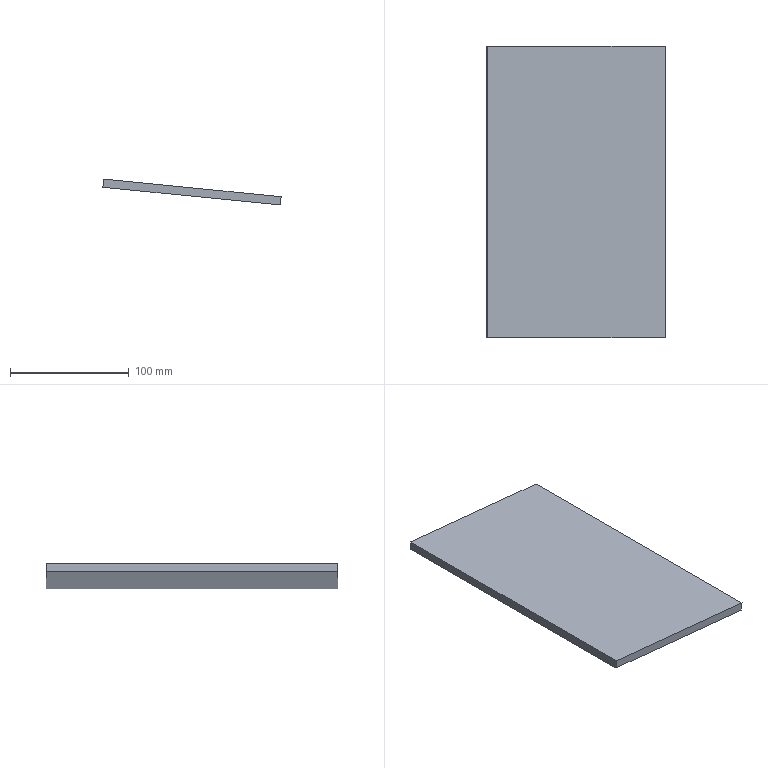Component | NX | MOVING_FRAME_BLOCK_2 | 1 solid | 6 faces | box 149.95 x 245 x 21.86 mm | volume 257250 mm3 | plane 6
STEP:
#1=CARTESIAN_POINT('',(0.,0.,0.));
#2=DIRECTION('',(0.,0.,1.));
#3=DIRECTION('',(1.,0.,0.));
#4=AXIS2_PLACEMENT_3D('',#1,#2,#3);
#5=CARTESIAN_POINT('',(837.5,1855.,424.634));
#6=VERTEX_POINT('',#5);
#7=CARTESIAN_POINT('',(838.195,1855.,431.599));
#8=VERTEX_POINT('',#7);
#9=CARTESIAN_POINT('',(837.5,1855.,424.634));
#10=DIRECTION('',(0.09932,0.,0.9951));
#11=VECTOR('',#10,1.);
#12=LINE('',#9,#11);
#13=CARTESIAN_POINT('',(837.5,1610.,424.634));
#14=DIRECTION('',(-0.9951,0.,0.09932));
#15=DIRECTION('',(-0.09932,0.,-0.9951));
#16=AXIS2_PLACEMENT_3D('',#13,#14,#15);
#17=PLANE('',#16);
#18=CARTESIAN_POINT('',(0.,-245.));
#19=DIRECTION('',(-1.,0.));
#20=VECTOR('',#19,1.);
#21=LINE('',#18,#20);
#22=(GEOMETRIC_REPRESENTATION_CONTEXT(2)PARAMETRIC_REPRESENTATION_CONTEXT()REPRESENTATION_CONTEXT('',''));
#23=DEFINITIONAL_REPRESENTATION('',(#21),#22);
#24=PCURVE('',#17,#23);
#25=CARTESIAN_POINT('',(838.195,1855.,431.599));
#26=DIRECTION('',(0.,1.,0.));
#27=DIRECTION('',(0.09932,0.,0.9951));
#28=AXIS2_PLACEMENT_3D('',#25,#26,#27);
#29=PLANE('',#28);
#30=CARTESIAN_POINT('',(-7.,-0.));
#31=DIRECTION('',(1.,0.));
#32=VECTOR('',#31,1.);
#33=LINE('',#30,#32);
#34=(GEOMETRIC_REPRESENTATION_CONTEXT(2)PARAMETRIC_REPRESENTATION_CONTEXT()REPRESENTATION_CONTEXT('',''));
#35=DEFINITIONAL_REPRESENTATION('',(#33),#34);
#36=PCURVE('',#29,#35);
#37=SURFACE_CURVE('',#12,(#24,#36),.PCURVE_S1.);
#38=EDGE_CURVE('',#6,#8,#37,.T.);
#39=ORIENTED_EDGE('',*,*,#38,.F.);
#40=CARTESIAN_POINT('',(837.5,1610.,424.634));
#41=VERTEX_POINT('',#40);
#42=CARTESIAN_POINT('',(837.5,1610.,424.634));
#43=DIRECTION('',(0.,1.,0.));
#44=VECTOR('',#43,1.);
#45=LINE('',#42,#44);
#46=CARTESIAN_POINT('',(0.,0.));
#47=DIRECTION('',(0.,-1.));
#48=VECTOR('',#47,1.);
#49=LINE('',#46,#48);
#50=(GEOMETRIC_REPRESENTATION_CONTEXT(2)PARAMETRIC_REPRESENTATION_CONTEXT()REPRESENTATION_CONTEXT('',''));
#51=DEFINITIONAL_REPRESENTATION('',(#49),#50);
#52=PCURVE('',#17,#51);
#53=CARTESIAN_POINT('',(986.758,1610.,409.736));
#54=DIRECTION('',(-0.09932,0.,-0.9951));
#55=DIRECTION('',(0.9951,0.,-0.09932));
#56=AXIS2_PLACEMENT_3D('',#53,#54,#55);
#57=PLANE('',#56);
#58=CARTESIAN_POINT('',(-150.,0.));
#59=DIRECTION('',(0.,-1.));
#60=VECTOR('',#59,1.);
#61=LINE('',#58,#60);
#62=(GEOMETRIC_REPRESENTATION_CONTEXT(2)PARAMETRIC_REPRESENTATION_CONTEXT()REPRESENTATION_CONTEXT('',''));
#63=DEFINITIONAL_REPRESENTATION('',(#61),#62);
#64=PCURVE('',#57,#63);
#65=SURFACE_CURVE('',#45,(#52,#64),.PCURVE_S1.);
#66=EDGE_CURVE('',#41,#6,#65,.T.);
#67=ORIENTED_EDGE('',*,*,#66,.F.);
#68=CARTESIAN_POINT('',(838.195,1610.,431.599));
#69=VERTEX_POINT('',#68);
#70=CARTESIAN_POINT('',(837.5,1610.,424.634));
#71=DIRECTION('',(0.09932,0.,0.9951));
#72=VECTOR('',#71,1.);
#73=LINE('',#70,#72);
#74=CARTESIAN_POINT('',(0.,0.));
#75=DIRECTION('',(-1.,0.));
#76=VECTOR('',#75,1.);
#77=LINE('',#74,#76);
#78=(GEOMETRIC_REPRESENTATION_CONTEXT(2)PARAMETRIC_REPRESENTATION_CONTEXT()REPRESENTATION_CONTEXT('',''));
#79=DEFINITIONAL_REPRESENTATION('',(#77),#78);
#80=PCURVE('',#17,#79);
#81=CARTESIAN_POINT('',(838.195,1610.,431.599));
#82=DIRECTION('',(0.,1.,0.));
#83=DIRECTION('',(0.09932,0.,0.9951));
#84=AXIS2_PLACEMENT_3D('',#81,#82,#83);
#85=PLANE('',#84);
#86=CARTESIAN_POINT('',(-7.,-0.));
#87=DIRECTION('',(1.,0.));
#88=VECTOR('',#87,1.);
#89=LINE('',#86,#88);
#90=(GEOMETRIC_REPRESENTATION_CONTEXT(2)PARAMETRIC_REPRESENTATION_CONTEXT()REPRESENTATION_CONTEXT('',''));
#91=DEFINITIONAL_REPRESENTATION('',(#89),#90);
#92=PCURVE('',#85,#91);
#93=SURFACE_CURVE('',#73,(#80,#92),.PCURVE_S1.);
#94=EDGE_CURVE('',#41,#69,#93,.T.);
#95=ORIENTED_EDGE('',*,*,#94,.T.);
#96=CARTESIAN_POINT('',(838.195,1610.,431.599));
#97=DIRECTION('',(0.,1.,0.));
#98=VECTOR('',#97,1.);
#99=LINE('',#96,#98);
#100=CARTESIAN_POINT('',(-7.,0.));
#101=DIRECTION('',(0.,-1.));
#102=VECTOR('',#101,1.);
#103=LINE('',#100,#102);
#104=(GEOMETRIC_REPRESENTATION_CONTEXT(2)PARAMETRIC_REPRESENTATION_CONTEXT()REPRESENTATION_CONTEXT('',''));
#105=DEFINITIONAL_REPRESENTATION('',(#103),#104);
#106=PCURVE('',#17,#105);
#107=CARTESIAN_POINT('',(838.195,1610.,431.599));
#108=DIRECTION('',(0.09932,0.,0.9951));
#109=DIRECTION('',(-0.9951,0.,0.09932));
#110=AXIS2_PLACEMENT_3D('',#107,#108,#109);
#111=PLANE('',#110);
#112=CARTESIAN_POINT('',(0.,0.));
#113=DIRECTION('',(0.,-1.));
#114=VECTOR('',#113,1.);
#115=LINE('',#112,#114);
#116=(GEOMETRIC_REPRESENTATION_CONTEXT(2)PARAMETRIC_REPRESENTATION_CONTEXT()REPRESENTATION_CONTEXT('',''));
#117=DEFINITIONAL_REPRESENTATION('',(#115),#116);
#118=PCURVE('',#111,#117);
#119=SURFACE_CURVE('',#99,(#106,#118),.PCURVE_S1.);
#120=EDGE_CURVE('',#69,#8,#119,.T.);
#121=ORIENTED_EDGE('',*,*,#120,.T.);
#122=EDGE_LOOP('',(#39,#67,#95,#121));
#123=FACE_BOUND('',#122,.T.);
#124=ADVANCED_FACE('',(#123),#17,.T.);
#125=CARTESIAN_POINT('',(987.454,1855.,416.701));
#126=VERTEX_POINT('',#125);
#127=CARTESIAN_POINT('',(838.195,1855.,431.599));
#128=DIRECTION('',(0.9951,0.,-0.09932));
#129=VECTOR('',#128,1.);
#130=LINE('',#127,#129);
#131=CARTESIAN_POINT('',(0.,-245.));
#132=DIRECTION('',(-1.,0.));
#133=VECTOR('',#132,1.);
#134=LINE('',#131,#133);
#135=(GEOMETRIC_REPRESENTATION_CONTEXT(2)PARAMETRIC_REPRESENTATION_CONTEXT()REPRESENTATION_CONTEXT('',''));
#136=DEFINITIONAL_REPRESENTATION('',(#134),#135);
#137=PCURVE('',#111,#136);
#138=CARTESIAN_POINT('',(0.,0.));
#139=DIRECTION('',(-0.,1.));
#140=VECTOR('',#139,1.);
#141=LINE('',#138,#140);
#142=(GEOMETRIC_REPRESENTATION_CONTEXT(2)PARAMETRIC_REPRESENTATION_CONTEXT()REPRESENTATION_CONTEXT('',''));
#143=DEFINITIONAL_REPRESENTATION('',(#141),#142);
#144=PCURVE('',#29,#143);
#145=SURFACE_CURVE('',#130,(#137,#144),.PCURVE_S1.);
#146=EDGE_CURVE('',#8,#126,#145,.T.);
#147=ORIENTED_EDGE('',*,*,#146,.F.);
#148=ORIENTED_EDGE('',*,*,#120,.F.);
#149=CARTESIAN_POINT('',(987.454,1610.,416.701));
#150=VERTEX_POINT('',#149);
#151=CARTESIAN_POINT('',(838.195,1610.,431.599));
#152=DIRECTION('',(0.9951,0.,-0.09932));
#153=VECTOR('',#152,1.);
#154=LINE('',#151,#153);
#155=CARTESIAN_POINT('',(0.,0.));
#156=DIRECTION('',(-1.,0.));
#157=VECTOR('',#156,1.);
#158=LINE('',#155,#157);
#159=(GEOMETRIC_REPRESENTATION_CONTEXT(2)PARAMETRIC_REPRESENTATION_CONTEXT()REPRESENTATION_CONTEXT('',''));
#160=DEFINITIONAL_REPRESENTATION('',(#158),#159);
#161=PCURVE('',#111,#160);
#162=CARTESIAN_POINT('',(0.,0.));
#163=DIRECTION('',(-0.,1.));
#164=VECTOR('',#163,1.);
#165=LINE('',#162,#164);
#166=(GEOMETRIC_REPRESENTATION_CONTEXT(2)PARAMETRIC_REPRESENTATION_CONTEXT()REPRESENTATION_CONTEXT('',''));
#167=DEFINITIONAL_REPRESENTATION('',(#165),#166);
#168=PCURVE('',#85,#167);
#169=SURFACE_CURVE('',#154,(#161,#168),.PCURVE_S1.);
#170=EDGE_CURVE('',#69,#150,#169,.T.);
#171=ORIENTED_EDGE('',*,*,#170,.T.);
#172=CARTESIAN_POINT('',(987.454,1610.,416.701));
#173=DIRECTION('',(0.,1.,0.));
#174=VECTOR('',#173,1.);
#175=LINE('',#172,#174);
#176=CARTESIAN_POINT('',(-150.,0.));
#177=DIRECTION('',(0.,-1.));
#178=VECTOR('',#177,1.);
#179=LINE('',#176,#178);
#180=(GEOMETRIC_REPRESENTATION_CONTEXT(2)PARAMETRIC_REPRESENTATION_CONTEXT()REPRESENTATION_CONTEXT('',''));
#181=DEFINITIONAL_REPRESENTATION('',(#179),#180);
#182=PCURVE('',#111,#181);
#183=CARTESIAN_POINT('',(987.454,1610.,416.701));
#184=DIRECTION('',(0.9951,0.,-0.09932));
#185=DIRECTION('',(0.09932,0.,0.9951));
#186=AXIS2_PLACEMENT_3D('',#183,#184,#185);
#187=PLANE('',#186);
#188=CARTESIAN_POINT('',(0.,0.));
#189=DIRECTION('',(0.,-1.));
#190=VECTOR('',#189,1.);
#191=LINE('',#188,#190);
#192=(GEOMETRIC_REPRESENTATION_CONTEXT(2)PARAMETRIC_REPRESENTATION_CONTEXT()REPRESENTATION_CONTEXT('',''));
#193=DEFINITIONAL_REPRESENTATION('',(#191),#192);
#194=PCURVE('',#187,#193);
#195=SURFACE_CURVE('',#175,(#182,#194),.PCURVE_S1.);
#196=EDGE_CURVE('',#150,#126,#195,.T.);
#197=ORIENTED_EDGE('',*,*,#196,.T.);
#198=EDGE_LOOP('',(#147,#148,#171,#197));
#199=FACE_BOUND('',#198,.T.);
#200=ADVANCED_FACE('',(#199),#111,.T.);
#201=CARTESIAN_POINT('',(986.758,1855.,409.736));
#202=VERTEX_POINT('',#201);
#203=CARTESIAN_POINT('',(987.454,1855.,416.701));
#204=DIRECTION('',(-0.09932,0.,-0.9951));
#205=VECTOR('',#204,1.);
#206=LINE('',#203,#205);
#207=CARTESIAN_POINT('',(0.,-245.));
#208=DIRECTION('',(-1.,0.));
#209=VECTOR('',#208,1.);
#210=LINE('',#207,#209);
#211=(GEOMETRIC_REPRESENTATION_CONTEXT(2)PARAMETRIC_REPRESENTATION_CONTEXT()REPRESENTATION_CONTEXT('',''));
#212=DEFINITIONAL_REPRESENTATION('',(#210),#211);
#213=PCURVE('',#187,#212);
#214=CARTESIAN_POINT('',(-0.,150.));
#215=DIRECTION('',(-1.,-0.));
#216=VECTOR('',#215,1.);
#217=LINE('',#214,#216);
#218=(GEOMETRIC_REPRESENTATION_CONTEXT(2)PARAMETRIC_REPRESENTATION_CONTEXT()REPRESENTATION_CONTEXT('',''));
#219=DEFINITIONAL_REPRESENTATION('',(#217),#218);
#220=PCURVE('',#29,#219);
#221=SURFACE_CURVE('',#206,(#213,#220),.PCURVE_S1.);
#222=EDGE_CURVE('',#126,#202,#221,.T.);
#223=ORIENTED_EDGE('',*,*,#222,.F.);
#224=ORIENTED_EDGE('',*,*,#196,.F.);
#225=CARTESIAN_POINT('',(986.758,1610.,409.736));
#226=VERTEX_POINT('',#225);
#227=CARTESIAN_POINT('',(987.454,1610.,416.701));
#228=DIRECTION('',(-0.09932,0.,-0.9951));
#229=VECTOR('',#228,1.);
#230=LINE('',#227,#229);
#231=CARTESIAN_POINT('',(0.,0.));
#232=DIRECTION('',(-1.,0.));
#233=VECTOR('',#232,1.);
#234=LINE('',#231,#233);
#235=(GEOMETRIC_REPRESENTATION_CONTEXT(2)PARAMETRIC_REPRESENTATION_CONTEXT()REPRESENTATION_CONTEXT('',''));
#236=DEFINITIONAL_REPRESENTATION('',(#234),#235);
#237=PCURVE('',#187,#236);
#238=CARTESIAN_POINT('',(-0.,150.));
#239=DIRECTION('',(-1.,-0.));
#240=VECTOR('',#239,1.);
#241=LINE('',#238,#240);
#242=(GEOMETRIC_REPRESENTATION_CONTEXT(2)PARAMETRIC_REPRESENTATION_CONTEXT()REPRESENTATION_CONTEXT('',''));
#243=DEFINITIONAL_REPRESENTATION('',(#241),#242);
#244=PCURVE('',#85,#243);
#245=SURFACE_CURVE('',#230,(#237,#244),.PCURVE_S1.);
#246=EDGE_CURVE('',#150,#226,#245,.T.);
#247=ORIENTED_EDGE('',*,*,#246,.T.);
#248=CARTESIAN_POINT('',(986.758,1610.,409.736));
#249=DIRECTION('',(0.,1.,0.));
#250=VECTOR('',#249,1.);
#251=LINE('',#248,#250);
#252=CARTESIAN_POINT('',(-7.,0.));
#253=DIRECTION('',(0.,-1.));
#254=VECTOR('',#253,1.);
#255=LINE('',#252,#254);
#256=(GEOMETRIC_REPRESENTATION_CONTEXT(2)PARAMETRIC_REPRESENTATION_CONTEXT()REPRESENTATION_CONTEXT('',''));
#257=DEFINITIONAL_REPRESENTATION('',(#255),#256);
#258=PCURVE('',#187,#257);
#259=CARTESIAN_POINT('',(0.,0.));
#260=DIRECTION('',(0.,-1.));
#261=VECTOR('',#260,1.);
#262=LINE('',#259,#261);
#263=(GEOMETRIC_REPRESENTATION_CONTEXT(2)PARAMETRIC_REPRESENTATION_CONTEXT()REPRESENTATION_CONTEXT('',''));
#264=DEFINITIONAL_REPRESENTATION('',(#262),#263);
#265=PCURVE('',#57,#264);
#266=SURFACE_CURVE('',#251,(#258,#265),.PCURVE_S1.);
#267=EDGE_CURVE('',#226,#202,#266,.T.);
#268=ORIENTED_EDGE('',*,*,#267,.T.);
#269=EDGE_LOOP('',(#223,#224,#247,#268));
#270=FACE_BOUND('',#269,.T.);
#271=ADVANCED_FACE('',(#270),#187,.T.);
#272=CARTESIAN_POINT('',(986.758,1855.,409.736));
#273=DIRECTION('',(-0.9951,0.,0.09932));
#274=VECTOR('',#273,1.);
#275=LINE('',#272,#274);
#276=CARTESIAN_POINT('',(0.,-245.));
#277=DIRECTION('',(-1.,0.));
#278=VECTOR('',#277,1.);
#279=LINE('',#276,#278);
#280=(GEOMETRIC_REPRESENTATION_CONTEXT(2)PARAMETRIC_REPRESENTATION_CONTEXT()REPRESENTATION_CONTEXT('',''));
#281=DEFINITIONAL_REPRESENTATION('',(#279),#280);
#282=PCURVE('',#57,#281);
#283=CARTESIAN_POINT('',(-7.,150.));
#284=DIRECTION('',(0.,-1.));
#285=VECTOR('',#284,1.);
#286=LINE('',#283,#285);
#287=(GEOMETRIC_REPRESENTATION_CONTEXT(2)PARAMETRIC_REPRESENTATION_CONTEXT()REPRESENTATION_CONTEXT('',''));
#288=DEFINITIONAL_REPRESENTATION('',(#286),#287);
#289=PCURVE('',#29,#288);
#290=SURFACE_CURVE('',#275,(#282,#289),.PCURVE_S1.);
#291=EDGE_CURVE('',#202,#6,#290,.T.);
#292=ORIENTED_EDGE('',*,*,#291,.F.);
#293=ORIENTED_EDGE('',*,*,#267,.F.);
#294=CARTESIAN_POINT('',(986.758,1610.,409.736));
#295=DIRECTION('',(-0.9951,0.,0.09932));
#296=VECTOR('',#295,1.);
#297=LINE('',#294,#296);
#298=CARTESIAN_POINT('',(0.,0.));
#299=DIRECTION('',(-1.,0.));
#300=VECTOR('',#299,1.);
#301=LINE('',#298,#300);
#302=(GEOMETRIC_REPRESENTATION_CONTEXT(2)PARAMETRIC_REPRESENTATION_CONTEXT()REPRESENTATION_CONTEXT('',''));
#303=DEFINITIONAL_REPRESENTATION('',(#301),#302);
#304=PCURVE('',#57,#303);
#305=CARTESIAN_POINT('',(-7.,150.));
#306=DIRECTION('',(0.,-1.));
#307=VECTOR('',#306,1.);
#308=LINE('',#305,#307);
#309=(GEOMETRIC_REPRESENTATION_CONTEXT(2)PARAMETRIC_REPRESENTATION_CONTEXT()REPRESENTATION_CONTEXT('',''));
#310=DEFINITIONAL_REPRESENTATION('',(#308),#309);
#311=PCURVE('',#85,#310);
#312=SURFACE_CURVE('',#297,(#304,#311),.PCURVE_S1.);
#313=EDGE_CURVE('',#226,#41,#312,.T.);
#314=ORIENTED_EDGE('',*,*,#313,.T.);
#315=ORIENTED_EDGE('',*,*,#66,.T.);
#316=EDGE_LOOP('',(#292,#293,#314,#315));
#317=FACE_BOUND('',#316,.T.);
#318=ADVANCED_FACE('',(#317),#57,.T.);
#319=ORIENTED_EDGE('',*,*,#94,.F.);
#320=ORIENTED_EDGE('',*,*,#313,.F.);
#321=ORIENTED_EDGE('',*,*,#246,.F.);
#322=ORIENTED_EDGE('',*,*,#170,.F.);
#323=EDGE_LOOP('',(#319,#320,#321,#322));
#324=FACE_BOUND('',#323,.T.);
#325=ADVANCED_FACE('',(#324),#85,.F.);
#326=ORIENTED_EDGE('',*,*,#38,.T.);
#327=ORIENTED_EDGE('',*,*,#146,.T.);
#328=ORIENTED_EDGE('',*,*,#222,.T.);
#329=ORIENTED_EDGE('',*,*,#291,.T.);
#330=EDGE_LOOP('',(#326,#327,#328,#329));
#331=FACE_BOUND('',#330,.T.);
#332=ADVANCED_FACE('',(#331),#29,.T.);
#333=CLOSED_SHELL('',(#124,#200,#271,#318,#325,#332));
#334=MANIFOLD_SOLID_BREP('',#333);
#335=(LENGTH_UNIT()NAMED_UNIT(*)SI_UNIT(.MILLI.,.METRE.));
#336=UNCERTAINTY_MEASURE_WITH_UNIT(LENGTH_MEASURE(0.0000001),#335,'','');
#337=(NAMED_UNIT(*)PLANE_ANGLE_UNIT()SI_UNIT($,.RADIAN.));
#338=(NAMED_UNIT(*)SI_UNIT($,.STERADIAN.)SOLID_ANGLE_UNIT());
#339=(GEOMETRIC_REPRESENTATION_CONTEXT(3)GLOBAL_UNCERTAINTY_ASSIGNED_CONTEXT((#336))GLOBAL_UNIT_ASSIGNED_CONTEXT((#335,#337,#338))REPRESENTATION_CONTEXT('',''));
#340=ADVANCED_BREP_SHAPE_REPRESENTATION('',(#4,#334),#339);